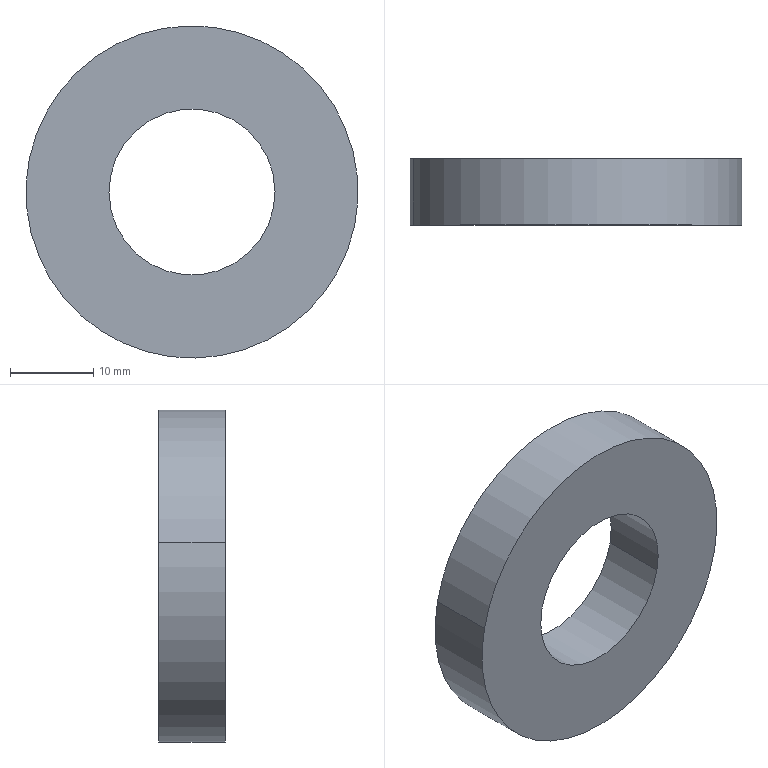Component | SolidWorks | 10-1 | 1 solid | 12 faces | box 40 x 8 x 40 mm | volume 4862 mm3 | cylinder 8 | plane 4 | commonest cylinder face diameters 40 x2 36 x2 26 x2 20 x2
build123d program:
from build123d import *


with BuildPart() as part:
    # Sketch1 → Revolve1 (revolve)
    with BuildSketch(Plane(origin=(0, 0, 0), x_dir=(1, 0, 0), z_dir=(0, 1, 0)), mode=Mode.PRIVATE) as revolve1_sk:
        Polygon((10, 0), (10, 8), (13, 8), (13, 2.5), (18, 2.5), (18, 8), (20, 8), (20, 0), align=None)
    revolve(revolve1_sk.sketch.rotate(Axis((0, 0, -25.37), (0, 0, 1)), 180), axis=Axis((0, 0, -25.37), (0, 0, 1)))


solid = part.part

# Placed as in the assembly
solid = solid.moved(Location((0, -73.702, 0), (90, 0, 0)))
STEP:
#1=COLOUR_RGB('',0.7922,0.8196,0.9333);
#2=FILL_AREA_STYLE_COLOUR('',#1);
#3=FILL_AREA_STYLE('',(#2));
#4=SURFACE_STYLE_FILL_AREA(#3);
#5=SURFACE_SIDE_STYLE('',(#4));
#6=SURFACE_STYLE_USAGE(.BOTH.,#5);
#7=PRESENTATION_STYLE_ASSIGNMENT((#6));
#8=CARTESIAN_POINT('',(-0.7712,-2.902,0.1589));
#9=VERTEX_POINT('',#8);
#10=CARTESIAN_POINT('',(0.7712,-2.902,-0.1589));
#11=VERTEX_POINT('',#10);
#12=CARTESIAN_POINT('',(-0.,-2.902,0.));
#13=DIRECTION('',(0.,1.,-0.));
#14=DIRECTION('',(-0.9794,0.,0.2018));
#15=AXIS2_PLACEMENT_3D('',#12,#13,#14);
#16=CIRCLE('',#15,0.7874);
#17=EDGE_CURVE('',#9,#11,#16,.T.);
#18=ORIENTED_EDGE('',*,*,#17,.T.);
#19=CARTESIAN_POINT('',(0.7712,-2.587,-0.1589));
#20=VERTEX_POINT('',#19);
#21=CARTESIAN_POINT('',(0.7712,-1.903,-0.1589));
#22=DIRECTION('',(0.,1.,-0.));
#23=VECTOR('',#22,39.37);
#24=LINE('',#21,#23);
#25=EDGE_CURVE('',#11,#20,#24,.T.);
#26=ORIENTED_EDGE('',*,*,#25,.T.);
#27=CARTESIAN_POINT('',(-0.7712,-2.587,0.1589));
#28=VERTEX_POINT('',#27);
#29=CARTESIAN_POINT('',(-0.,-2.587,0.));
#30=DIRECTION('',(0.,1.,-0.));
#31=DIRECTION('',(-0.9794,0.,0.2018));
#32=AXIS2_PLACEMENT_3D('',#29,#30,#31);
#33=CIRCLE('',#32,0.7874);
#34=EDGE_CURVE('',#28,#20,#33,.T.);
#35=ORIENTED_EDGE('',*,*,#34,.F.);
#36=CARTESIAN_POINT('',(-0.7712,-1.903,0.1589));
#37=DIRECTION('',(0.,1.,-0.));
#38=VECTOR('',#37,39.37);
#39=LINE('',#36,#38);
#40=EDGE_CURVE('',#9,#28,#39,.T.);
#41=ORIENTED_EDGE('',*,*,#40,.F.);
#42=EDGE_LOOP('',(#18,#26,#35,#41));
#43=FACE_OUTER_BOUND('',#42,.T.);
#44=CARTESIAN_POINT('',(-0.,-1.903,0.));
#45=DIRECTION('',(0.,1.,-0.));
#46=DIRECTION('',(-0.9794,0.,0.2018));
#47=AXIS2_PLACEMENT_3D('',#44,#45,#46);
#48=CYLINDRICAL_SURFACE('',#47,0.7874);
#49=ADVANCED_FACE('',(#43),#48,.T.);
#50=CARTESIAN_POINT('',(0.6941,-2.803,-0.143));
#51=VERTEX_POINT('',#50);
#52=CARTESIAN_POINT('',(-0.6941,-2.803,0.143));
#53=VERTEX_POINT('',#52);
#54=CARTESIAN_POINT('',(-0.,-2.803,0.));
#55=DIRECTION('',(0.,1.,-0.));
#56=DIRECTION('',(-0.9794,0.,0.2018));
#57=AXIS2_PLACEMENT_3D('',#54,#55,#56);
#58=CIRCLE('',#57,0.7087);
#59=EDGE_CURVE('',#51,#53,#58,.T.);
#60=ORIENTED_EDGE('',*,*,#59,.F.);
#61=CARTESIAN_POINT('',(0.6941,-2.587,-0.143));
#62=VERTEX_POINT('',#61);
#63=CARTESIAN_POINT('',(0.6941,-1.903,-0.143));
#64=DIRECTION('',(0.,1.,-0.));
#65=VECTOR('',#64,39.37);
#66=LINE('',#63,#65);
#67=EDGE_CURVE('',#51,#62,#66,.T.);
#68=ORIENTED_EDGE('',*,*,#67,.T.);
#69=CARTESIAN_POINT('',(-0.6941,-2.587,0.143));
#70=VERTEX_POINT('',#69);
#71=CARTESIAN_POINT('',(-0.,-2.587,0.));
#72=DIRECTION('',(0.,1.,-0.));
#73=DIRECTION('',(-0.9794,0.,0.2018));
#74=AXIS2_PLACEMENT_3D('',#71,#72,#73);
#75=CIRCLE('',#74,0.7087);
#76=EDGE_CURVE('',#62,#70,#75,.T.);
#77=ORIENTED_EDGE('',*,*,#76,.T.);
#78=CARTESIAN_POINT('',(-0.6941,-1.903,0.143));
#79=DIRECTION('',(0.,1.,-0.));
#80=VECTOR('',#79,39.37);
#81=LINE('',#78,#80);
#82=EDGE_CURVE('',#53,#70,#81,.T.);
#83=ORIENTED_EDGE('',*,*,#82,.F.);
#84=EDGE_LOOP('',(#60,#68,#77,#83));
#85=FACE_OUTER_BOUND('',#84,.T.);
#86=CARTESIAN_POINT('',(-0.,-1.903,0.));
#87=DIRECTION('',(0.,1.,-0.));
#88=DIRECTION('',(-0.9794,0.,0.2018));
#89=AXIS2_PLACEMENT_3D('',#86,#87,#88);
#90=CYLINDRICAL_SURFACE('',#89,0.7087);
#91=ADVANCED_FACE('',(#85),#90,.F.);
#92=CARTESIAN_POINT('',(-0.5013,-2.803,0.1033));
#93=VERTEX_POINT('',#92);
#94=CARTESIAN_POINT('',(0.5013,-2.803,-0.1033));
#95=VERTEX_POINT('',#94);
#96=CARTESIAN_POINT('',(-0.,-2.803,0.));
#97=DIRECTION('',(0.,1.,-0.));
#98=DIRECTION('',(-0.9794,0.,0.2018));
#99=AXIS2_PLACEMENT_3D('',#96,#97,#98);
#100=CIRCLE('',#99,0.5118);
#101=EDGE_CURVE('',#93,#95,#100,.T.);
#102=ORIENTED_EDGE('',*,*,#101,.T.);
#103=CARTESIAN_POINT('',(0.5013,-2.587,-0.1033));
#104=VERTEX_POINT('',#103);
#105=CARTESIAN_POINT('',(0.5013,-1.903,-0.1033));
#106=DIRECTION('',(0.,1.,-0.));
#107=VECTOR('',#106,39.37);
#108=LINE('',#105,#107);
#109=EDGE_CURVE('',#95,#104,#108,.T.);
#110=ORIENTED_EDGE('',*,*,#109,.T.);
#111=CARTESIAN_POINT('',(-0.5013,-2.587,0.1033));
#112=VERTEX_POINT('',#111);
#113=CARTESIAN_POINT('',(-0.,-2.587,0.));
#114=DIRECTION('',(0.,1.,-0.));
#115=DIRECTION('',(-0.9794,0.,0.2018));
#116=AXIS2_PLACEMENT_3D('',#113,#114,#115);
#117=CIRCLE('',#116,0.5118);
#118=EDGE_CURVE('',#112,#104,#117,.T.);
#119=ORIENTED_EDGE('',*,*,#118,.F.);
#120=CARTESIAN_POINT('',(-0.5013,-1.903,0.1033));
#121=DIRECTION('',(0.,1.,-0.));
#122=VECTOR('',#121,39.37);
#123=LINE('',#120,#122);
#124=EDGE_CURVE('',#93,#112,#123,.T.);
#125=ORIENTED_EDGE('',*,*,#124,.F.);
#126=EDGE_LOOP('',(#102,#110,#119,#125));
#127=FACE_OUTER_BOUND('',#126,.T.);
#128=CARTESIAN_POINT('',(-0.,-1.903,0.));
#129=DIRECTION('',(0.,1.,-0.));
#130=DIRECTION('',(-0.9794,0.,0.2018));
#131=AXIS2_PLACEMENT_3D('',#128,#129,#130);
#132=CYLINDRICAL_SURFACE('',#131,0.5118);
#133=ADVANCED_FACE('',(#127),#132,.T.);
#134=CARTESIAN_POINT('',(0.3856,-2.902,-0.07946));
#135=VERTEX_POINT('',#134);
#136=CARTESIAN_POINT('',(-0.3856,-2.902,0.07946));
#137=VERTEX_POINT('',#136);
#138=CARTESIAN_POINT('',(-0.,-2.902,0.));
#139=DIRECTION('',(0.,1.,-0.));
#140=DIRECTION('',(-0.9794,0.,0.2018));
#141=AXIS2_PLACEMENT_3D('',#138,#139,#140);
#142=CIRCLE('',#141,0.3937);
#143=EDGE_CURVE('',#135,#137,#142,.T.);
#144=ORIENTED_EDGE('',*,*,#143,.F.);
#145=CARTESIAN_POINT('',(0.3856,-2.587,-0.07946));
#146=VERTEX_POINT('',#145);
#147=CARTESIAN_POINT('',(0.3856,-1.903,-0.07946));
#148=DIRECTION('',(0.,1.,-0.));
#149=VECTOR('',#148,39.37);
#150=LINE('',#147,#149);
#151=EDGE_CURVE('',#135,#146,#150,.T.);
#152=ORIENTED_EDGE('',*,*,#151,.T.);
#153=CARTESIAN_POINT('',(-0.3856,-2.587,0.07946));
#154=VERTEX_POINT('',#153);
#155=CARTESIAN_POINT('',(-0.,-2.587,0.));
#156=DIRECTION('',(0.,1.,-0.));
#157=DIRECTION('',(-0.9794,0.,0.2018));
#158=AXIS2_PLACEMENT_3D('',#155,#156,#157);
#159=CIRCLE('',#158,0.3937);
#160=EDGE_CURVE('',#146,#154,#159,.T.);
#161=ORIENTED_EDGE('',*,*,#160,.T.);
#162=CARTESIAN_POINT('',(-0.3856,-1.903,0.07946));
#163=DIRECTION('',(0.,1.,-0.));
#164=VECTOR('',#163,39.37);
#165=LINE('',#162,#164);
#166=EDGE_CURVE('',#137,#154,#165,.T.);
#167=ORIENTED_EDGE('',*,*,#166,.F.);
#168=EDGE_LOOP('',(#144,#152,#161,#167));
#169=FACE_OUTER_BOUND('',#168,.T.);
#170=CARTESIAN_POINT('',(-0.,-1.903,0.));
#171=DIRECTION('',(0.,1.,-0.));
#172=DIRECTION('',(-0.9794,0.,0.2018));
#173=AXIS2_PLACEMENT_3D('',#170,#171,#172);
#174=CYLINDRICAL_SURFACE('',#173,0.3937);
#175=ADVANCED_FACE('',(#169),#174,.F.);
#176=ORIENTED_EDGE('',*,*,#17,.F.);
#177=CARTESIAN_POINT('',(-0.,-2.902,0.));
#178=DIRECTION('',(0.,1.,-0.));
#179=DIRECTION('',(-0.9794,0.,0.2018));
#180=AXIS2_PLACEMENT_3D('',#177,#178,#179);
#181=CIRCLE('',#180,0.7874);
#182=EDGE_CURVE('',#11,#9,#181,.T.);
#183=ORIENTED_EDGE('',*,*,#182,.F.);
#184=EDGE_LOOP('',(#176,#183));
#185=FACE_OUTER_BOUND('',#184,.T.);
#186=CARTESIAN_POINT('',(-0.,-2.902,0.));
#187=DIRECTION('',(0.,1.,-0.));
#188=DIRECTION('',(-0.9794,0.,0.2018));
#189=AXIS2_PLACEMENT_3D('',#186,#187,#188);
#190=CIRCLE('',#189,0.3937);
#191=EDGE_CURVE('',#137,#135,#190,.T.);
#192=ORIENTED_EDGE('',*,*,#191,.T.);
#193=ORIENTED_EDGE('',*,*,#143,.T.);
#194=EDGE_LOOP('',(#192,#193));
#195=FACE_BOUND('',#194,.T.);
#196=CARTESIAN_POINT('',(0.7712,-2.902,-0.1589));
#197=DIRECTION('',(0.,1.,-0.));
#198=DIRECTION('',(-0.9794,0.,0.2018));
#199=AXIS2_PLACEMENT_3D('',#196,#197,#198);
#200=PLANE('',#199);
#201=ADVANCED_FACE('',(#185,#195),#200,.F.);
#202=ORIENTED_EDGE('',*,*,#151,.F.);
#203=ORIENTED_EDGE('',*,*,#191,.F.);
#204=ORIENTED_EDGE('',*,*,#166,.T.);
#205=CARTESIAN_POINT('',(-0.,-2.587,0.));
#206=DIRECTION('',(0.,1.,-0.));
#207=DIRECTION('',(-0.9794,0.,0.2018));
#208=AXIS2_PLACEMENT_3D('',#205,#206,#207);
#209=CIRCLE('',#208,0.3937);
#210=EDGE_CURVE('',#154,#146,#209,.T.);
#211=ORIENTED_EDGE('',*,*,#210,.T.);
#212=EDGE_LOOP('',(#202,#203,#204,#211));
#213=FACE_OUTER_BOUND('',#212,.T.);
#214=CARTESIAN_POINT('',(-0.,-1.903,0.));
#215=DIRECTION('',(0.,1.,-0.));
#216=DIRECTION('',(-0.9794,0.,0.2018));
#217=AXIS2_PLACEMENT_3D('',#214,#215,#216);
#218=CYLINDRICAL_SURFACE('',#217,0.3937);
#219=ADVANCED_FACE('',(#213),#218,.F.);
#220=ORIENTED_EDGE('',*,*,#210,.F.);
#221=ORIENTED_EDGE('',*,*,#160,.F.);
#222=EDGE_LOOP('',(#220,#221));
#223=FACE_BOUND('',#222,.T.);
#224=ORIENTED_EDGE('',*,*,#118,.T.);
#225=CARTESIAN_POINT('',(-0.,-2.587,0.));
#226=DIRECTION('',(0.,1.,-0.));
#227=DIRECTION('',(-0.9794,0.,0.2018));
#228=AXIS2_PLACEMENT_3D('',#225,#226,#227);
#229=CIRCLE('',#228,0.5118);
#230=EDGE_CURVE('',#104,#112,#229,.T.);
#231=ORIENTED_EDGE('',*,*,#230,.T.);
#232=EDGE_LOOP('',(#224,#231));
#233=FACE_OUTER_BOUND('',#232,.T.);
#234=CARTESIAN_POINT('',(0.3856,-2.587,-0.07946));
#235=DIRECTION('',(-0.,-1.,0.));
#236=DIRECTION('',(0.9794,-0.,-0.2018));
#237=AXIS2_PLACEMENT_3D('',#234,#235,#236);
#238=PLANE('',#237);
#239=ADVANCED_FACE('',(#223,#233),#238,.F.);
#240=ORIENTED_EDGE('',*,*,#109,.F.);
#241=CARTESIAN_POINT('',(-0.,-2.803,0.));
#242=DIRECTION('',(0.,1.,-0.));
#243=DIRECTION('',(-0.9794,0.,0.2018));
#244=AXIS2_PLACEMENT_3D('',#241,#242,#243);
#245=CIRCLE('',#244,0.5118);
#246=EDGE_CURVE('',#95,#93,#245,.T.);
#247=ORIENTED_EDGE('',*,*,#246,.T.);
#248=ORIENTED_EDGE('',*,*,#124,.T.);
#249=ORIENTED_EDGE('',*,*,#230,.F.);
#250=EDGE_LOOP('',(#240,#247,#248,#249));
#251=FACE_OUTER_BOUND('',#250,.T.);
#252=CARTESIAN_POINT('',(-0.,-1.903,0.));
#253=DIRECTION('',(0.,1.,-0.));
#254=DIRECTION('',(-0.9794,0.,0.2018));
#255=AXIS2_PLACEMENT_3D('',#252,#253,#254);
#256=CYLINDRICAL_SURFACE('',#255,0.5118);
#257=ADVANCED_FACE('',(#251),#256,.T.);
#258=ORIENTED_EDGE('',*,*,#101,.F.);
#259=ORIENTED_EDGE('',*,*,#246,.F.);
#260=EDGE_LOOP('',(#258,#259));
#261=FACE_BOUND('',#260,.T.);
#262=CARTESIAN_POINT('',(-0.,-2.803,0.));
#263=DIRECTION('',(0.,1.,-0.));
#264=DIRECTION('',(-0.9794,0.,0.2018));
#265=AXIS2_PLACEMENT_3D('',#262,#263,#264);
#266=CIRCLE('',#265,0.7087);
#267=EDGE_CURVE('',#53,#51,#266,.T.);
#268=ORIENTED_EDGE('',*,*,#267,.T.);
#269=ORIENTED_EDGE('',*,*,#59,.T.);
#270=EDGE_LOOP('',(#268,#269));
#271=FACE_OUTER_BOUND('',#270,.T.);
#272=CARTESIAN_POINT('',(0.5013,-2.803,-0.1033));
#273=DIRECTION('',(-0.,-1.,0.));
#274=DIRECTION('',(0.9794,-0.,-0.2018));
#275=AXIS2_PLACEMENT_3D('',#272,#273,#274);
#276=PLANE('',#275);
#277=ADVANCED_FACE('',(#261,#271),#276,.F.);
#278=ORIENTED_EDGE('',*,*,#67,.F.);
#279=ORIENTED_EDGE('',*,*,#267,.F.);
#280=ORIENTED_EDGE('',*,*,#82,.T.);
#281=CARTESIAN_POINT('',(-0.,-2.587,0.));
#282=DIRECTION('',(0.,1.,-0.));
#283=DIRECTION('',(-0.9794,0.,0.2018));
#284=AXIS2_PLACEMENT_3D('',#281,#282,#283);
#285=CIRCLE('',#284,0.7087);
#286=EDGE_CURVE('',#70,#62,#285,.T.);
#287=ORIENTED_EDGE('',*,*,#286,.T.);
#288=EDGE_LOOP('',(#278,#279,#280,#287));
#289=FACE_OUTER_BOUND('',#288,.T.);
#290=CARTESIAN_POINT('',(-0.,-1.903,0.));
#291=DIRECTION('',(0.,1.,-0.));
#292=DIRECTION('',(-0.9794,0.,0.2018));
#293=AXIS2_PLACEMENT_3D('',#290,#291,#292);
#294=CYLINDRICAL_SURFACE('',#293,0.7087);
#295=ADVANCED_FACE('',(#289),#294,.F.);
#296=ORIENTED_EDGE('',*,*,#286,.F.);
#297=ORIENTED_EDGE('',*,*,#76,.F.);
#298=EDGE_LOOP('',(#296,#297));
#299=FACE_BOUND('',#298,.T.);
#300=ORIENTED_EDGE('',*,*,#34,.T.);
#301=CARTESIAN_POINT('',(-0.,-2.587,0.));
#302=DIRECTION('',(0.,1.,-0.));
#303=DIRECTION('',(-0.9794,0.,0.2018));
#304=AXIS2_PLACEMENT_3D('',#301,#302,#303);
#305=CIRCLE('',#304,0.7874);
#306=EDGE_CURVE('',#20,#28,#305,.T.);
#307=ORIENTED_EDGE('',*,*,#306,.T.);
#308=EDGE_LOOP('',(#300,#307));
#309=FACE_OUTER_BOUND('',#308,.T.);
#310=CARTESIAN_POINT('',(0.6941,-2.587,-0.143));
#311=DIRECTION('',(-0.,-1.,0.));
#312=DIRECTION('',(0.9794,-0.,-0.2018));
#313=AXIS2_PLACEMENT_3D('',#310,#311,#312);
#314=PLANE('',#313);
#315=ADVANCED_FACE('',(#299,#309),#314,.F.);
#316=ORIENTED_EDGE('',*,*,#25,.F.);
#317=ORIENTED_EDGE('',*,*,#182,.T.);
#318=ORIENTED_EDGE('',*,*,#40,.T.);
#319=ORIENTED_EDGE('',*,*,#306,.F.);
#320=EDGE_LOOP('',(#316,#317,#318,#319));
#321=FACE_OUTER_BOUND('',#320,.T.);
#322=CARTESIAN_POINT('',(-0.,-1.903,0.));
#323=DIRECTION('',(0.,1.,-0.));
#324=DIRECTION('',(-0.9794,0.,0.2018));
#325=AXIS2_PLACEMENT_3D('',#322,#323,#324);
#326=CYLINDRICAL_SURFACE('',#325,0.7874);
#327=ADVANCED_FACE('',(#321),#326,.T.);
#328=CLOSED_SHELL('',(#49,#91,#133,#175,#201,#219,#239,#257,#277,#295,#315,#327));
#329=MANIFOLD_SOLID_BREP('',#328);
#330=STYLED_ITEM('',(#7),#329);
#331=(LENGTH_UNIT()NAMED_UNIT(*)SI_UNIT($,.METRE.));
#332=LENGTH_MEASURE_WITH_UNIT(LENGTH_MEASURE(0.0254),#331);
#333=DIMENSIONAL_EXPONENTS(1.,0.,0.,0.,0.,0.,0.);
#334=(CONVERSION_BASED_UNIT('',#332)LENGTH_UNIT()NAMED_UNIT(#333));
#335=UNCERTAINTY_MEASURE_WITH_UNIT(LENGTH_MEASURE(0.00001),#334,'','');
#336=(NAMED_UNIT(*)PLANE_ANGLE_UNIT()SI_UNIT($,.RADIAN.));
#337=(NAMED_UNIT(*)SI_UNIT($,.STERADIAN.)SOLID_ANGLE_UNIT());
#338=(GEOMETRIC_REPRESENTATION_CONTEXT(3)GLOBAL_UNCERTAINTY_ASSIGNED_CONTEXT((#335))GLOBAL_UNIT_ASSIGNED_CONTEXT((#334,#336,#337))REPRESENTATION_CONTEXT('',''));
#339=MECHANICAL_DESIGN_GEOMETRIC_PRESENTATION_REPRESENTATION('',(#330),#338);
#340=CARTESIAN_POINT('',(0.,0.,0.));
#341=DIRECTION('',(0.,0.,1.));
#342=DIRECTION('',(1.,0.,0.));
#343=AXIS2_PLACEMENT_3D('',#340,#341,#342);
#344=(LENGTH_UNIT()NAMED_UNIT(*)SI_UNIT($,.METRE.));
#345=LENGTH_MEASURE_WITH_UNIT(LENGTH_MEASURE(0.0254),#344);
#346=DIMENSIONAL_EXPONENTS(1.,0.,0.,0.,0.,0.,0.);
#347=(CONVERSION_BASED_UNIT('',#345)LENGTH_UNIT()NAMED_UNIT(#346));
#348=UNCERTAINTY_MEASURE_WITH_UNIT(LENGTH_MEASURE(0.00001),#347,'','');
#349=(NAMED_UNIT(*)PLANE_ANGLE_UNIT()SI_UNIT($,.RADIAN.));
#350=(NAMED_UNIT(*)SI_UNIT($,.STERADIAN.)SOLID_ANGLE_UNIT());
#351=(GEOMETRIC_REPRESENTATION_CONTEXT(3)GLOBAL_UNCERTAINTY_ASSIGNED_CONTEXT((#348))GLOBAL_UNIT_ASSIGNED_CONTEXT((#347,#349,#350))REPRESENTATION_CONTEXT('',''));
#352=ADVANCED_BREP_SHAPE_REPRESENTATION('',(#329,#343),#351);
#353=PRESENTATION_LAYER_ASSIGNMENT('','',(#330));